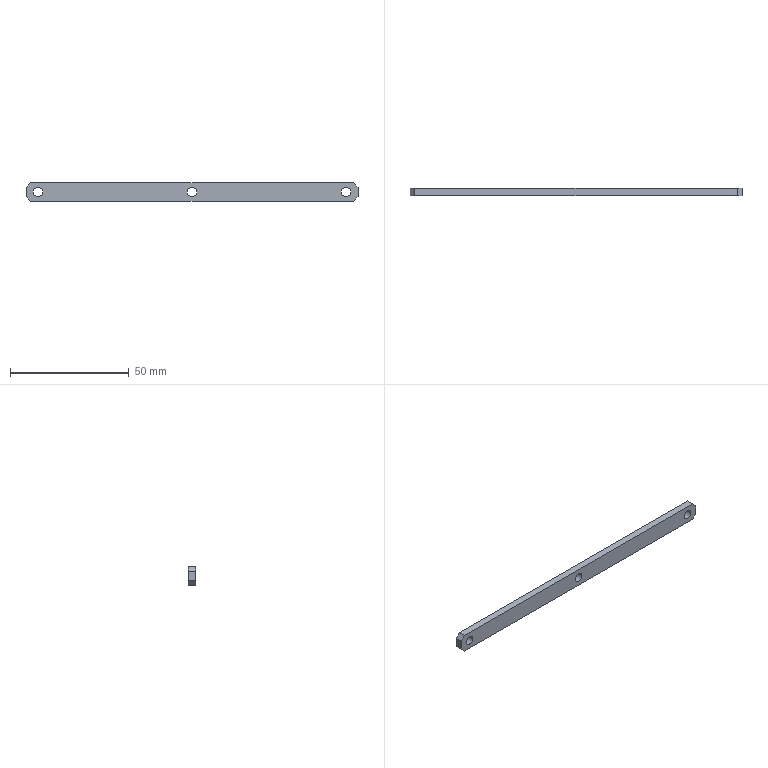Component | SolidWorks | MTCTV2104DJ006-000-0004LimitStrip-1 | 1 solid | 16 faces | box 140 x 3 x 8 mm | volume 3223 mm3 | plane 10 | cylinder 6 | commonest cylinder face diameters 4 x6
build123d program:
from build123d import *

# Parameters (mm, degrees)
SKETCH1_W                = 140
SKETCH1_H                = 8
BOSS_EXTRUDE1_DEPTH      = 3
CHAMFER1_SIZE            = 2
F_4_0_4_DIAMETER_HOLE1_D = 4


with BuildPart() as part:
    # Sketch1 → Boss-Extrude1 (new body)
    with BuildSketch(Plane(origin=(0, 0, 0), x_dir=(0, 0, -1), z_dir=(1, 0, 0))):
        Rectangle(SKETCH1_W, SKETCH1_H)
    extrude(amount=BOSS_EXTRUDE1_DEPTH)

    # Chamfer1
    chamfer1_edges = [part.edges().sort_by_distance(p)[0] for p in [
        (1.5, -4, -70),
        (1.5, -4, 70),
        (1.5, 4, 70),
        (1.5, 4, -70),
    ]]
    chamfer(chamfer1_edges, length=CHAMFER1_SIZE)

    # 4.0 _4_ Diameter Hole1 (through all)
    with Locations(Plane(origin=(3, 0, 0), x_dir=(0, 0, -1), z_dir=(1, 0, 0))):
        with Locations((0, 0), (-65, 0), (65, 0)):
            Hole(F_4_0_4_DIAMETER_HOLE1_D / 2)


solid = part.part

# Placed as in the assembly
solid = solid.moved(Location((-122.536, 39.25, 217.788), (90, -90, 0)))
STEP:
#1=COLOUR_RGB('',0.7922,0.8196,0.9333);
#2=FILL_AREA_STYLE_COLOUR('',#1);
#3=FILL_AREA_STYLE('',(#2));
#4=SURFACE_STYLE_FILL_AREA(#3);
#5=SURFACE_SIDE_STYLE('',(#4));
#6=SURFACE_STYLE_USAGE(.BOTH.,#5);
#7=PRESENTATION_STYLE_ASSIGNMENT((#6));
#8=CARTESIAN_POINT('',(-4.903,1.427,8.574));
#9=VERTEX_POINT('',#8);
#10=CARTESIAN_POINT('',(-4.746,1.427,8.574));
#11=VERTEX_POINT('',#10);
#12=CARTESIAN_POINT('',(-4.824,1.427,8.574));
#13=DIRECTION('',(-0.,1.,0.));
#14=DIRECTION('',(1.,0.,0.));
#15=AXIS2_PLACEMENT_3D('',#12,#13,#14);
#16=CIRCLE('',#15,0.07874);
#17=EDGE_CURVE('',#9,#11,#16,.T.);
#18=ORIENTED_EDGE('',*,*,#17,.F.);
#19=CARTESIAN_POINT('',(-4.903,1.545,8.574));
#20=VERTEX_POINT('',#19);
#21=CARTESIAN_POINT('',(-4.903,1.545,8.574));
#22=DIRECTION('',(-0.,1.,0.));
#23=VECTOR('',#22,39.37);
#24=LINE('',#21,#23);
#25=EDGE_CURVE('',#9,#20,#24,.T.);
#26=ORIENTED_EDGE('',*,*,#25,.T.);
#27=CARTESIAN_POINT('',(-4.746,1.545,8.574));
#28=VERTEX_POINT('',#27);
#29=CARTESIAN_POINT('',(-4.824,1.545,8.574));
#30=DIRECTION('',(-0.,1.,0.));
#31=DIRECTION('',(1.,0.,0.));
#32=AXIS2_PLACEMENT_3D('',#29,#30,#31);
#33=CIRCLE('',#32,0.07874);
#34=EDGE_CURVE('',#20,#28,#33,.T.);
#35=ORIENTED_EDGE('',*,*,#34,.T.);
#36=CARTESIAN_POINT('',(-4.746,1.545,8.574));
#37=DIRECTION('',(-0.,1.,0.));
#38=VECTOR('',#37,39.37);
#39=LINE('',#36,#38);
#40=EDGE_CURVE('',#11,#28,#39,.T.);
#41=ORIENTED_EDGE('',*,*,#40,.F.);
#42=EDGE_LOOP('',(#18,#26,#35,#41));
#43=FACE_OUTER_BOUND('',#42,.T.);
#44=CARTESIAN_POINT('',(-4.824,1.545,8.574));
#45=DIRECTION('',(-0.,1.,0.));
#46=DIRECTION('',(1.,0.,0.));
#47=AXIS2_PLACEMENT_3D('',#44,#45,#46);
#48=CYLINDRICAL_SURFACE('',#47,0.07874);
#49=ADVANCED_FACE('',(#43),#48,.F.);
#50=CARTESIAN_POINT('',(-7.462,1.427,8.574));
#51=VERTEX_POINT('',#50);
#52=CARTESIAN_POINT('',(-7.305,1.427,8.574));
#53=VERTEX_POINT('',#52);
#54=CARTESIAN_POINT('',(-7.383,1.427,8.574));
#55=DIRECTION('',(-0.,1.,0.));
#56=DIRECTION('',(1.,0.,0.));
#57=AXIS2_PLACEMENT_3D('',#54,#55,#56);
#58=CIRCLE('',#57,0.07874);
#59=EDGE_CURVE('',#51,#53,#58,.T.);
#60=ORIENTED_EDGE('',*,*,#59,.F.);
#61=CARTESIAN_POINT('',(-7.462,1.545,8.574));
#62=VERTEX_POINT('',#61);
#63=CARTESIAN_POINT('',(-7.462,1.545,8.574));
#64=DIRECTION('',(-0.,1.,0.));
#65=VECTOR('',#64,39.37);
#66=LINE('',#63,#65);
#67=EDGE_CURVE('',#51,#62,#66,.T.);
#68=ORIENTED_EDGE('',*,*,#67,.T.);
#69=CARTESIAN_POINT('',(-7.305,1.545,8.574));
#70=VERTEX_POINT('',#69);
#71=CARTESIAN_POINT('',(-7.383,1.545,8.574));
#72=DIRECTION('',(-0.,1.,0.));
#73=DIRECTION('',(1.,0.,0.));
#74=AXIS2_PLACEMENT_3D('',#71,#72,#73);
#75=CIRCLE('',#74,0.07874);
#76=EDGE_CURVE('',#62,#70,#75,.T.);
#77=ORIENTED_EDGE('',*,*,#76,.T.);
#78=CARTESIAN_POINT('',(-7.305,1.545,8.574));
#79=DIRECTION('',(-0.,1.,0.));
#80=VECTOR('',#79,39.37);
#81=LINE('',#78,#80);
#82=EDGE_CURVE('',#53,#70,#81,.T.);
#83=ORIENTED_EDGE('',*,*,#82,.F.);
#84=EDGE_LOOP('',(#60,#68,#77,#83));
#85=FACE_OUTER_BOUND('',#84,.T.);
#86=CARTESIAN_POINT('',(-7.383,1.545,8.574));
#87=DIRECTION('',(-0.,1.,0.));
#88=DIRECTION('',(1.,0.,0.));
#89=AXIS2_PLACEMENT_3D('',#86,#87,#88);
#90=CYLINDRICAL_SURFACE('',#89,0.07874);
#91=ADVANCED_FACE('',(#85),#90,.F.);
#92=CARTESIAN_POINT('',(-2.344,1.427,8.574));
#93=VERTEX_POINT('',#92);
#94=CARTESIAN_POINT('',(-2.186,1.427,8.574));
#95=VERTEX_POINT('',#94);
#96=CARTESIAN_POINT('',(-2.265,1.427,8.574));
#97=DIRECTION('',(-0.,1.,0.));
#98=DIRECTION('',(1.,0.,0.));
#99=AXIS2_PLACEMENT_3D('',#96,#97,#98);
#100=CIRCLE('',#99,0.07874);
#101=EDGE_CURVE('',#93,#95,#100,.T.);
#102=ORIENTED_EDGE('',*,*,#101,.F.);
#103=CARTESIAN_POINT('',(-2.344,1.545,8.574));
#104=VERTEX_POINT('',#103);
#105=CARTESIAN_POINT('',(-2.344,1.545,8.574));
#106=DIRECTION('',(-0.,1.,0.));
#107=VECTOR('',#106,39.37);
#108=LINE('',#105,#107);
#109=EDGE_CURVE('',#93,#104,#108,.T.);
#110=ORIENTED_EDGE('',*,*,#109,.T.);
#111=CARTESIAN_POINT('',(-2.186,1.545,8.574));
#112=VERTEX_POINT('',#111);
#113=CARTESIAN_POINT('',(-2.265,1.545,8.574));
#114=DIRECTION('',(-0.,1.,0.));
#115=DIRECTION('',(1.,0.,0.));
#116=AXIS2_PLACEMENT_3D('',#113,#114,#115);
#117=CIRCLE('',#116,0.07874);
#118=EDGE_CURVE('',#104,#112,#117,.T.);
#119=ORIENTED_EDGE('',*,*,#118,.T.);
#120=CARTESIAN_POINT('',(-2.186,1.545,8.574));
#121=DIRECTION('',(-0.,1.,0.));
#122=VECTOR('',#121,39.37);
#123=LINE('',#120,#122);
#124=EDGE_CURVE('',#95,#112,#123,.T.);
#125=ORIENTED_EDGE('',*,*,#124,.F.);
#126=EDGE_LOOP('',(#102,#110,#119,#125));
#127=FACE_OUTER_BOUND('',#126,.T.);
#128=CARTESIAN_POINT('',(-2.265,1.545,8.574));
#129=DIRECTION('',(-0.,1.,0.));
#130=DIRECTION('',(1.,0.,0.));
#131=AXIS2_PLACEMENT_3D('',#128,#129,#130);
#132=CYLINDRICAL_SURFACE('',#131,0.07874);
#133=ADVANCED_FACE('',(#127),#132,.F.);
#134=CARTESIAN_POINT('',(-2.068,1.427,8.653));
#135=VERTEX_POINT('',#134);
#136=CARTESIAN_POINT('',(-2.068,1.427,8.496));
#137=VERTEX_POINT('',#136);
#138=CARTESIAN_POINT('',(-2.068,1.427,8.732));
#139=DIRECTION('',(0.,0.,-1.));
#140=VECTOR('',#139,39.37);
#141=LINE('',#138,#140);
#142=EDGE_CURVE('',#135,#137,#141,.T.);
#143=ORIENTED_EDGE('',*,*,#142,.T.);
#144=CARTESIAN_POINT('',(-2.068,1.545,8.496));
#145=VERTEX_POINT('',#144);
#146=CARTESIAN_POINT('',(-2.068,1.545,8.496));
#147=DIRECTION('',(-0.,1.,0.));
#148=VECTOR('',#147,39.37);
#149=LINE('',#146,#148);
#150=EDGE_CURVE('',#137,#145,#149,.T.);
#151=ORIENTED_EDGE('',*,*,#150,.T.);
#152=CARTESIAN_POINT('',(-2.068,1.545,8.653));
#153=VERTEX_POINT('',#152);
#154=CARTESIAN_POINT('',(-2.068,1.545,8.732));
#155=DIRECTION('',(0.,0.,-1.));
#156=VECTOR('',#155,39.37);
#157=LINE('',#154,#156);
#158=EDGE_CURVE('',#153,#145,#157,.T.);
#159=ORIENTED_EDGE('',*,*,#158,.F.);
#160=CARTESIAN_POINT('',(-2.068,1.545,8.653));
#161=DIRECTION('',(0.,-1.,-0.));
#162=VECTOR('',#161,39.37);
#163=LINE('',#160,#162);
#164=EDGE_CURVE('',#153,#135,#163,.T.);
#165=ORIENTED_EDGE('',*,*,#164,.T.);
#166=EDGE_LOOP('',(#143,#151,#159,#165));
#167=FACE_OUTER_BOUND('',#166,.T.);
#168=CARTESIAN_POINT('',(-2.068,1.545,8.732));
#169=DIRECTION('',(-1.,-0.,-0.));
#170=DIRECTION('',(-0.,1.,0.));
#171=AXIS2_PLACEMENT_3D('',#168,#169,#170);
#172=PLANE('',#171);
#173=ADVANCED_FACE('',(#167),#172,.F.);
#174=CARTESIAN_POINT('',(-2.147,1.545,8.417));
#175=VERTEX_POINT('',#174);
#176=CARTESIAN_POINT('',(-7.501,1.545,8.417));
#177=VERTEX_POINT('',#176);
#178=CARTESIAN_POINT('',(-7.58,1.545,8.417));
#179=DIRECTION('',(-1.,-0.,-0.));
#180=VECTOR('',#179,39.37);
#181=LINE('',#178,#180);
#182=EDGE_CURVE('',#175,#177,#181,.T.);
#183=ORIENTED_EDGE('',*,*,#182,.F.);
#184=CARTESIAN_POINT('',(-2.147,1.427,8.417));
#185=VERTEX_POINT('',#184);
#186=CARTESIAN_POINT('',(-2.147,1.545,8.417));
#187=DIRECTION('',(0.,-1.,-0.));
#188=VECTOR('',#187,39.37);
#189=LINE('',#186,#188);
#190=EDGE_CURVE('',#175,#185,#189,.T.);
#191=ORIENTED_EDGE('',*,*,#190,.T.);
#192=CARTESIAN_POINT('',(-7.501,1.427,8.417));
#193=VERTEX_POINT('',#192);
#194=CARTESIAN_POINT('',(-7.58,1.427,8.417));
#195=DIRECTION('',(-1.,-0.,-0.));
#196=VECTOR('',#195,39.37);
#197=LINE('',#194,#196);
#198=EDGE_CURVE('',#185,#193,#197,.T.);
#199=ORIENTED_EDGE('',*,*,#198,.T.);
#200=CARTESIAN_POINT('',(-7.501,1.545,8.417));
#201=DIRECTION('',(-0.,1.,0.));
#202=VECTOR('',#201,39.37);
#203=LINE('',#200,#202);
#204=EDGE_CURVE('',#193,#177,#203,.T.);
#205=ORIENTED_EDGE('',*,*,#204,.T.);
#206=EDGE_LOOP('',(#183,#191,#199,#205));
#207=FACE_OUTER_BOUND('',#206,.T.);
#208=CARTESIAN_POINT('',(-7.58,1.545,8.417));
#209=DIRECTION('',(-0.,-0.,1.));
#210=DIRECTION('',(1.,0.,0.));
#211=AXIS2_PLACEMENT_3D('',#208,#209,#210);
#212=PLANE('',#211);
#213=ADVANCED_FACE('',(#207),#212,.F.);
#214=CARTESIAN_POINT('',(-7.58,1.427,8.496));
#215=VERTEX_POINT('',#214);
#216=CARTESIAN_POINT('',(-7.58,1.427,8.653));
#217=VERTEX_POINT('',#216);
#218=CARTESIAN_POINT('',(-7.58,1.427,8.732));
#219=DIRECTION('',(-0.,-0.,1.));
#220=VECTOR('',#219,39.37);
#221=LINE('',#218,#220);
#222=EDGE_CURVE('',#215,#217,#221,.T.);
#223=ORIENTED_EDGE('',*,*,#222,.T.);
#224=CARTESIAN_POINT('',(-7.58,1.545,8.653));
#225=VERTEX_POINT('',#224);
#226=CARTESIAN_POINT('',(-7.58,1.545,8.653));
#227=DIRECTION('',(-0.,1.,0.));
#228=VECTOR('',#227,39.37);
#229=LINE('',#226,#228);
#230=EDGE_CURVE('',#217,#225,#229,.T.);
#231=ORIENTED_EDGE('',*,*,#230,.T.);
#232=CARTESIAN_POINT('',(-7.58,1.545,8.496));
#233=VERTEX_POINT('',#232);
#234=CARTESIAN_POINT('',(-7.58,1.545,8.732));
#235=DIRECTION('',(-0.,-0.,1.));
#236=VECTOR('',#235,39.37);
#237=LINE('',#234,#236);
#238=EDGE_CURVE('',#233,#225,#237,.T.);
#239=ORIENTED_EDGE('',*,*,#238,.F.);
#240=CARTESIAN_POINT('',(-7.58,1.545,8.496));
#241=DIRECTION('',(0.,-1.,-0.));
#242=VECTOR('',#241,39.37);
#243=LINE('',#240,#242);
#244=EDGE_CURVE('',#233,#215,#243,.T.);
#245=ORIENTED_EDGE('',*,*,#244,.T.);
#246=EDGE_LOOP('',(#223,#231,#239,#245));
#247=FACE_OUTER_BOUND('',#246,.T.);
#248=CARTESIAN_POINT('',(-7.58,1.545,8.732));
#249=DIRECTION('',(1.,0.,0.));
#250=DIRECTION('',(0.,-1.,-0.));
#251=AXIS2_PLACEMENT_3D('',#248,#249,#250);
#252=PLANE('',#251);
#253=ADVANCED_FACE('',(#247),#252,.F.);
#254=CARTESIAN_POINT('',(-7.501,1.427,8.732));
#255=VERTEX_POINT('',#254);
#256=CARTESIAN_POINT('',(-2.147,1.427,8.732));
#257=VERTEX_POINT('',#256);
#258=CARTESIAN_POINT('',(-7.58,1.427,8.732));
#259=DIRECTION('',(1.,0.,0.));
#260=VECTOR('',#259,39.37);
#261=LINE('',#258,#260);
#262=EDGE_CURVE('',#255,#257,#261,.T.);
#263=ORIENTED_EDGE('',*,*,#262,.T.);
#264=CARTESIAN_POINT('',(-2.147,1.545,8.732));
#265=VERTEX_POINT('',#264);
#266=CARTESIAN_POINT('',(-2.147,1.545,8.732));
#267=DIRECTION('',(-0.,1.,0.));
#268=VECTOR('',#267,39.37);
#269=LINE('',#266,#268);
#270=EDGE_CURVE('',#257,#265,#269,.T.);
#271=ORIENTED_EDGE('',*,*,#270,.T.);
#272=CARTESIAN_POINT('',(-7.501,1.545,8.732));
#273=VERTEX_POINT('',#272);
#274=CARTESIAN_POINT('',(-7.58,1.545,8.732));
#275=DIRECTION('',(1.,0.,0.));
#276=VECTOR('',#275,39.37);
#277=LINE('',#274,#276);
#278=EDGE_CURVE('',#273,#265,#277,.T.);
#279=ORIENTED_EDGE('',*,*,#278,.F.);
#280=CARTESIAN_POINT('',(-7.501,1.545,8.732));
#281=DIRECTION('',(0.,-1.,-0.));
#282=VECTOR('',#281,39.37);
#283=LINE('',#280,#282);
#284=EDGE_CURVE('',#273,#255,#283,.T.);
#285=ORIENTED_EDGE('',*,*,#284,.T.);
#286=EDGE_LOOP('',(#263,#271,#279,#285));
#287=FACE_OUTER_BOUND('',#286,.T.);
#288=CARTESIAN_POINT('',(-7.58,1.545,8.732));
#289=DIRECTION('',(0.,0.,-1.));
#290=DIRECTION('',(-1.,-0.,-0.));
#291=AXIS2_PLACEMENT_3D('',#288,#289,#290);
#292=PLANE('',#291);
#293=ADVANCED_FACE('',(#287),#292,.F.);
#294=CARTESIAN_POINT('',(-4.824,1.545,8.574));
#295=DIRECTION('',(-0.,1.,0.));
#296=DIRECTION('',(1.,0.,0.));
#297=AXIS2_PLACEMENT_3D('',#294,#295,#296);
#298=CIRCLE('',#297,0.07874);
#299=EDGE_CURVE('',#28,#20,#298,.T.);
#300=ORIENTED_EDGE('',*,*,#299,.F.);
#301=ORIENTED_EDGE('',*,*,#34,.F.);
#302=EDGE_LOOP('',(#300,#301));
#303=FACE_BOUND('',#302,.T.);
#304=CARTESIAN_POINT('',(-7.383,1.545,8.574));
#305=DIRECTION('',(-0.,1.,0.));
#306=DIRECTION('',(1.,0.,0.));
#307=AXIS2_PLACEMENT_3D('',#304,#305,#306);
#308=CIRCLE('',#307,0.07874);
#309=EDGE_CURVE('',#70,#62,#308,.T.);
#310=ORIENTED_EDGE('',*,*,#309,.F.);
#311=ORIENTED_EDGE('',*,*,#76,.F.);
#312=EDGE_LOOP('',(#310,#311));
#313=FACE_BOUND('',#312,.T.);
#314=CARTESIAN_POINT('',(-2.265,1.545,8.574));
#315=DIRECTION('',(-0.,1.,0.));
#316=DIRECTION('',(1.,0.,0.));
#317=AXIS2_PLACEMENT_3D('',#314,#315,#316);
#318=CIRCLE('',#317,0.07874);
#319=EDGE_CURVE('',#112,#104,#318,.T.);
#320=ORIENTED_EDGE('',*,*,#319,.F.);
#321=ORIENTED_EDGE('',*,*,#118,.F.);
#322=EDGE_LOOP('',(#320,#321));
#323=FACE_BOUND('',#322,.T.);
#324=ORIENTED_EDGE('',*,*,#158,.T.);
#325=CARTESIAN_POINT('',(-2.147,1.545,8.417));
#326=DIRECTION('',(-0.7071,0.,-0.7071));
#327=VECTOR('',#326,39.37);
#328=LINE('',#325,#327);
#329=EDGE_CURVE('',#145,#175,#328,.T.);
#330=ORIENTED_EDGE('',*,*,#329,.T.);
#331=ORIENTED_EDGE('',*,*,#182,.T.);
#332=CARTESIAN_POINT('',(-7.58,1.545,8.496));
#333=DIRECTION('',(-0.7071,-0.,0.7071));
#334=VECTOR('',#333,39.37);
#335=LINE('',#332,#334);
#336=EDGE_CURVE('',#177,#233,#335,.T.);
#337=ORIENTED_EDGE('',*,*,#336,.T.);
#338=ORIENTED_EDGE('',*,*,#238,.T.);
#339=CARTESIAN_POINT('',(-7.501,1.545,8.732));
#340=DIRECTION('',(0.7071,-0.,0.7071));
#341=VECTOR('',#340,39.37);
#342=LINE('',#339,#341);
#343=EDGE_CURVE('',#225,#273,#342,.T.);
#344=ORIENTED_EDGE('',*,*,#343,.T.);
#345=ORIENTED_EDGE('',*,*,#278,.T.);
#346=CARTESIAN_POINT('',(-2.068,1.545,8.653));
#347=DIRECTION('',(0.7071,0.,-0.7071));
#348=VECTOR('',#347,39.37);
#349=LINE('',#346,#348);
#350=EDGE_CURVE('',#265,#153,#349,.T.);
#351=ORIENTED_EDGE('',*,*,#350,.T.);
#352=EDGE_LOOP('',(#324,#330,#331,#337,#338,#344,#345,#351));
#353=FACE_OUTER_BOUND('',#352,.T.);
#354=CARTESIAN_POINT('',(-4.824,1.545,8.574));
#355=DIRECTION('',(0.,-1.,-0.));
#356=DIRECTION('',(-1.,-0.,-0.));
#357=AXIS2_PLACEMENT_3D('',#354,#355,#356);
#358=PLANE('',#357);
#359=ADVANCED_FACE('',(#303,#313,#323,#353),#358,.F.);
#360=CARTESIAN_POINT('',(-4.824,1.427,8.574));
#361=DIRECTION('',(-0.,1.,0.));
#362=DIRECTION('',(1.,0.,0.));
#363=AXIS2_PLACEMENT_3D('',#360,#361,#362);
#364=CIRCLE('',#363,0.07874);
#365=EDGE_CURVE('',#11,#9,#364,.T.);
#366=ORIENTED_EDGE('',*,*,#365,.T.);
#367=ORIENTED_EDGE('',*,*,#17,.T.);
#368=EDGE_LOOP('',(#366,#367));
#369=FACE_BOUND('',#368,.T.);
#370=CARTESIAN_POINT('',(-7.383,1.427,8.574));
#371=DIRECTION('',(-0.,1.,0.));
#372=DIRECTION('',(1.,0.,0.));
#373=AXIS2_PLACEMENT_3D('',#370,#371,#372);
#374=CIRCLE('',#373,0.07874);
#375=EDGE_CURVE('',#53,#51,#374,.T.);
#376=ORIENTED_EDGE('',*,*,#375,.T.);
#377=ORIENTED_EDGE('',*,*,#59,.T.);
#378=EDGE_LOOP('',(#376,#377));
#379=FACE_BOUND('',#378,.T.);
#380=CARTESIAN_POINT('',(-2.265,1.427,8.574));
#381=DIRECTION('',(-0.,1.,0.));
#382=DIRECTION('',(1.,0.,0.));
#383=AXIS2_PLACEMENT_3D('',#380,#381,#382);
#384=CIRCLE('',#383,0.07874);
#385=EDGE_CURVE('',#95,#93,#384,.T.);
#386=ORIENTED_EDGE('',*,*,#385,.T.);
#387=ORIENTED_EDGE('',*,*,#101,.T.);
#388=EDGE_LOOP('',(#386,#387));
#389=FACE_BOUND('',#388,.T.);
#390=ORIENTED_EDGE('',*,*,#198,.F.);
#391=CARTESIAN_POINT('',(-3.407,1.427,7.157));
#392=DIRECTION('',(0.7071,-0.,0.7071));
#393=VECTOR('',#392,39.37);
#394=LINE('',#391,#393);
#395=EDGE_CURVE('',#185,#137,#394,.T.);
#396=ORIENTED_EDGE('',*,*,#395,.T.);
#397=ORIENTED_EDGE('',*,*,#142,.F.);
#398=CARTESIAN_POINT('',(-3.407,1.427,9.992));
#399=DIRECTION('',(-0.7071,-0.,0.7071));
#400=VECTOR('',#399,39.37);
#401=LINE('',#398,#400);
#402=EDGE_CURVE('',#135,#257,#401,.T.);
#403=ORIENTED_EDGE('',*,*,#402,.T.);
#404=ORIENTED_EDGE('',*,*,#262,.F.);
#405=CARTESIAN_POINT('',(-6.242,1.427,9.992));
#406=DIRECTION('',(-0.7071,0.,-0.7071));
#407=VECTOR('',#406,39.37);
#408=LINE('',#405,#407);
#409=EDGE_CURVE('',#255,#217,#408,.T.);
#410=ORIENTED_EDGE('',*,*,#409,.T.);
#411=ORIENTED_EDGE('',*,*,#222,.F.);
#412=CARTESIAN_POINT('',(-6.242,1.427,7.157));
#413=DIRECTION('',(0.7071,0.,-0.7071));
#414=VECTOR('',#413,39.37);
#415=LINE('',#412,#414);
#416=EDGE_CURVE('',#215,#193,#415,.T.);
#417=ORIENTED_EDGE('',*,*,#416,.T.);
#418=EDGE_LOOP('',(#390,#396,#397,#403,#404,#410,#411,#417));
#419=FACE_OUTER_BOUND('',#418,.T.);
#420=CARTESIAN_POINT('',(-4.824,1.427,8.574));
#421=DIRECTION('',(0.,-1.,-0.));
#422=DIRECTION('',(-1.,-0.,-0.));
#423=AXIS2_PLACEMENT_3D('',#420,#421,#422);
#424=PLANE('',#423);
#425=ADVANCED_FACE('',(#369,#379,#389,#419),#424,.T.);
#426=ORIENTED_EDGE('',*,*,#329,.F.);
#427=ORIENTED_EDGE('',*,*,#150,.F.);
#428=ORIENTED_EDGE('',*,*,#395,.F.);
#429=ORIENTED_EDGE('',*,*,#190,.F.);
#430=EDGE_LOOP('',(#426,#427,#428,#429));
#431=FACE_OUTER_BOUND('',#430,.T.);
#432=CARTESIAN_POINT('',(-2.147,1.545,8.417));
#433=DIRECTION('',(-0.7071,-0.,0.7071));
#434=DIRECTION('',(0.,-1.,-0.));
#435=AXIS2_PLACEMENT_3D('',#432,#433,#434);
#436=PLANE('',#435);
#437=ADVANCED_FACE('',(#431),#436,.F.);
#438=ORIENTED_EDGE('',*,*,#350,.F.);
#439=ORIENTED_EDGE('',*,*,#270,.F.);
#440=ORIENTED_EDGE('',*,*,#402,.F.);
#441=ORIENTED_EDGE('',*,*,#164,.F.);
#442=EDGE_LOOP('',(#438,#439,#440,#441));
#443=FACE_OUTER_BOUND('',#442,.T.);
#444=CARTESIAN_POINT('',(-2.068,1.545,8.653));
#445=DIRECTION('',(-0.7071,0.,-0.7071));
#446=DIRECTION('',(0.,-1.,-0.));
#447=AXIS2_PLACEMENT_3D('',#444,#445,#446);
#448=PLANE('',#447);
#449=ADVANCED_FACE('',(#443),#448,.F.);
#450=ORIENTED_EDGE('',*,*,#343,.F.);
#451=ORIENTED_EDGE('',*,*,#230,.F.);
#452=ORIENTED_EDGE('',*,*,#409,.F.);
#453=ORIENTED_EDGE('',*,*,#284,.F.);
#454=EDGE_LOOP('',(#450,#451,#452,#453));
#455=FACE_OUTER_BOUND('',#454,.T.);
#456=CARTESIAN_POINT('',(-7.501,1.545,8.732));
#457=DIRECTION('',(0.7071,0.,-0.7071));
#458=DIRECTION('',(0.,-1.,-0.));
#459=AXIS2_PLACEMENT_3D('',#456,#457,#458);
#460=PLANE('',#459);
#461=ADVANCED_FACE('',(#455),#460,.F.);
#462=ORIENTED_EDGE('',*,*,#336,.F.);
#463=ORIENTED_EDGE('',*,*,#204,.F.);
#464=ORIENTED_EDGE('',*,*,#416,.F.);
#465=ORIENTED_EDGE('',*,*,#244,.F.);
#466=EDGE_LOOP('',(#462,#463,#464,#465));
#467=FACE_OUTER_BOUND('',#466,.T.);
#468=CARTESIAN_POINT('',(-7.58,1.545,8.496));
#469=DIRECTION('',(0.7071,-0.,0.7071));
#470=DIRECTION('',(0.,-1.,-0.));
#471=AXIS2_PLACEMENT_3D('',#468,#469,#470);
#472=PLANE('',#471);
#473=ADVANCED_FACE('',(#467),#472,.F.);
#474=ORIENTED_EDGE('',*,*,#109,.F.);
#475=ORIENTED_EDGE('',*,*,#385,.F.);
#476=ORIENTED_EDGE('',*,*,#124,.T.);
#477=ORIENTED_EDGE('',*,*,#319,.T.);
#478=EDGE_LOOP('',(#474,#475,#476,#477));
#479=FACE_OUTER_BOUND('',#478,.T.);
#480=CARTESIAN_POINT('',(-2.265,1.545,8.574));
#481=DIRECTION('',(-0.,1.,0.));
#482=DIRECTION('',(1.,0.,0.));
#483=AXIS2_PLACEMENT_3D('',#480,#481,#482);
#484=CYLINDRICAL_SURFACE('',#483,0.07874);
#485=ADVANCED_FACE('',(#479),#484,.F.);
#486=ORIENTED_EDGE('',*,*,#67,.F.);
#487=ORIENTED_EDGE('',*,*,#375,.F.);
#488=ORIENTED_EDGE('',*,*,#82,.T.);
#489=ORIENTED_EDGE('',*,*,#309,.T.);
#490=EDGE_LOOP('',(#486,#487,#488,#489));
#491=FACE_OUTER_BOUND('',#490,.T.);
#492=CARTESIAN_POINT('',(-7.383,1.545,8.574));
#493=DIRECTION('',(-0.,1.,0.));
#494=DIRECTION('',(1.,0.,0.));
#495=AXIS2_PLACEMENT_3D('',#492,#493,#494);
#496=CYLINDRICAL_SURFACE('',#495,0.07874);
#497=ADVANCED_FACE('',(#491),#496,.F.);
#498=ORIENTED_EDGE('',*,*,#25,.F.);
#499=ORIENTED_EDGE('',*,*,#365,.F.);
#500=ORIENTED_EDGE('',*,*,#40,.T.);
#501=ORIENTED_EDGE('',*,*,#299,.T.);
#502=EDGE_LOOP('',(#498,#499,#500,#501));
#503=FACE_OUTER_BOUND('',#502,.T.);
#504=CARTESIAN_POINT('',(-4.824,1.545,8.574));
#505=DIRECTION('',(-0.,1.,0.));
#506=DIRECTION('',(1.,0.,0.));
#507=AXIS2_PLACEMENT_3D('',#504,#505,#506);
#508=CYLINDRICAL_SURFACE('',#507,0.07874);
#509=ADVANCED_FACE('',(#503),#508,.F.);
#510=CLOSED_SHELL('',(#49,#91,#133,#173,#213,#253,#293,#359,#425,#437,#449,#461,#473,#485,#497,#509));
#511=MANIFOLD_SOLID_BREP('',#510);
#512=STYLED_ITEM('',(#7),#511);
#513=PRESENTATION_LAYER_ASSIGNMENT('','',(#512));
#514=CARTESIAN_POINT('',(0.,0.,0.));
#515=DIRECTION('',(0.,0.,1.));
#516=DIRECTION('',(1.,0.,0.));
#517=AXIS2_PLACEMENT_3D('',#514,#515,#516);
#518=(LENGTH_UNIT()NAMED_UNIT(*)SI_UNIT($,.METRE.));
#519=LENGTH_MEASURE_WITH_UNIT(LENGTH_MEASURE(0.0254),#518);
#520=DIMENSIONAL_EXPONENTS(1.,0.,0.,0.,0.,0.,0.);
#521=(CONVERSION_BASED_UNIT('',#519)LENGTH_UNIT()NAMED_UNIT(#520));
#522=UNCERTAINTY_MEASURE_WITH_UNIT(LENGTH_MEASURE(0.00001),#521,'','');
#523=(NAMED_UNIT(*)PLANE_ANGLE_UNIT()SI_UNIT($,.RADIAN.));
#524=(NAMED_UNIT(*)SI_UNIT($,.STERADIAN.)SOLID_ANGLE_UNIT());
#525=(GEOMETRIC_REPRESENTATION_CONTEXT(3)GLOBAL_UNCERTAINTY_ASSIGNED_CONTEXT((#522))GLOBAL_UNIT_ASSIGNED_CONTEXT((#521,#523,#524))REPRESENTATION_CONTEXT('',''));
#526=ADVANCED_BREP_SHAPE_REPRESENTATION('',(#511,#517),#525);
#527=(LENGTH_UNIT()NAMED_UNIT(*)SI_UNIT($,.METRE.));
#528=LENGTH_MEASURE_WITH_UNIT(LENGTH_MEASURE(0.0254),#527);
#529=DIMENSIONAL_EXPONENTS(1.,0.,0.,0.,0.,0.,0.);
#530=(CONVERSION_BASED_UNIT('',#528)LENGTH_UNIT()NAMED_UNIT(#529));
#531=UNCERTAINTY_MEASURE_WITH_UNIT(LENGTH_MEASURE(0.00001),#530,'','');
#532=(NAMED_UNIT(*)PLANE_ANGLE_UNIT()SI_UNIT($,.RADIAN.));
#533=(NAMED_UNIT(*)SI_UNIT($,.STERADIAN.)SOLID_ANGLE_UNIT());
#534=(GEOMETRIC_REPRESENTATION_CONTEXT(3)GLOBAL_UNCERTAINTY_ASSIGNED_CONTEXT((#531))GLOBAL_UNIT_ASSIGNED_CONTEXT((#530,#532,#533))REPRESENTATION_CONTEXT('',''));
#535=MECHANICAL_DESIGN_GEOMETRIC_PRESENTATION_REPRESENTATION('',(#512),#534);